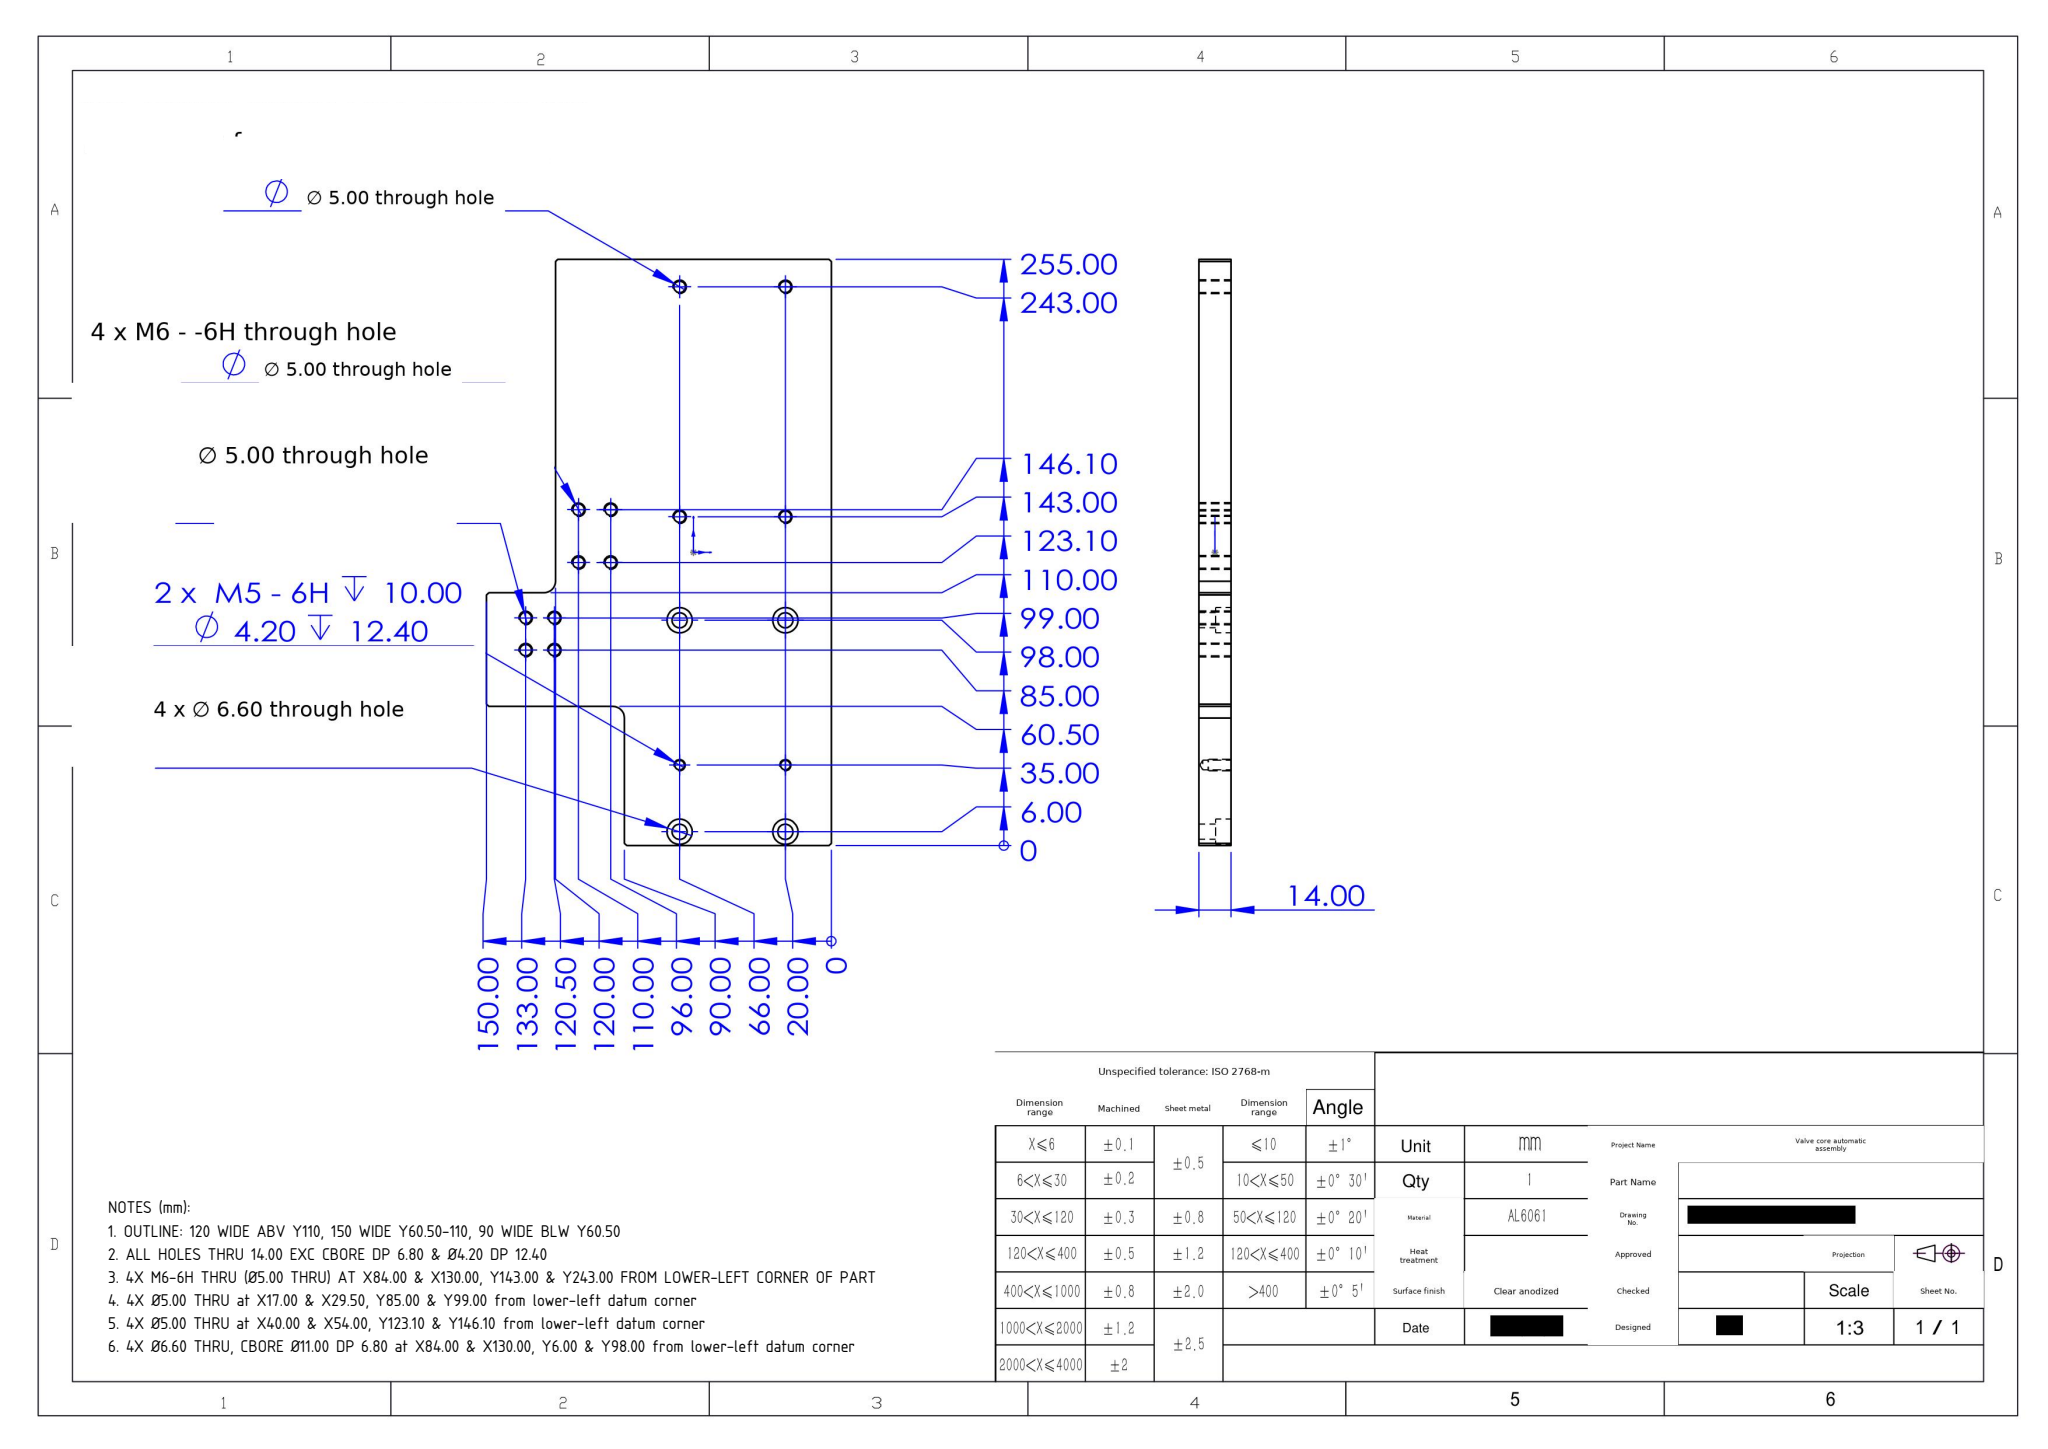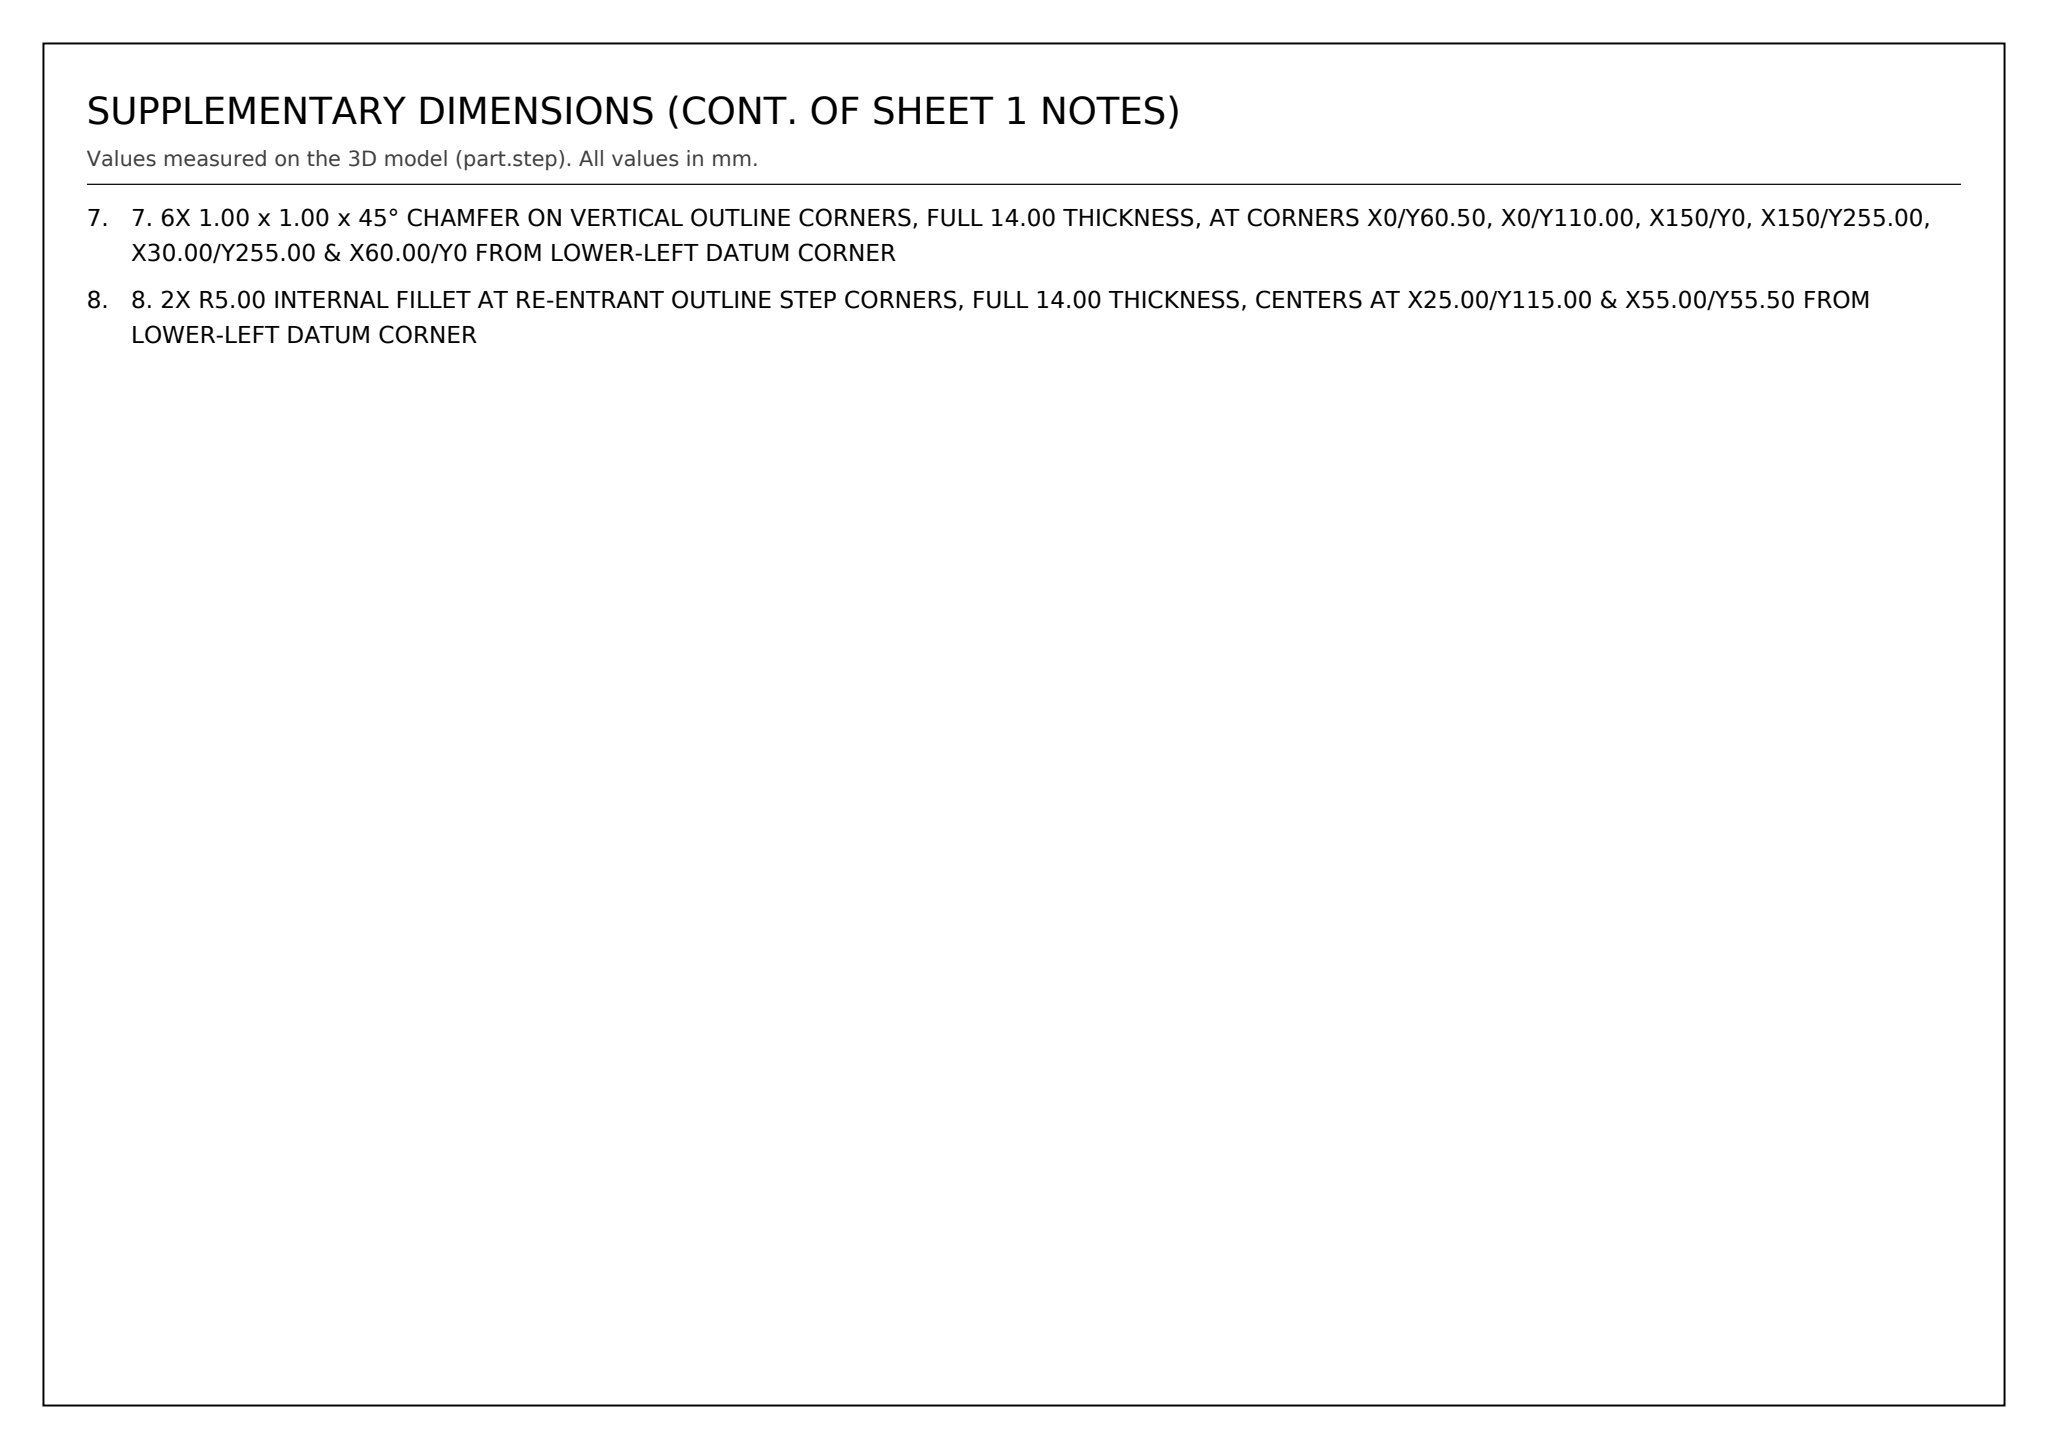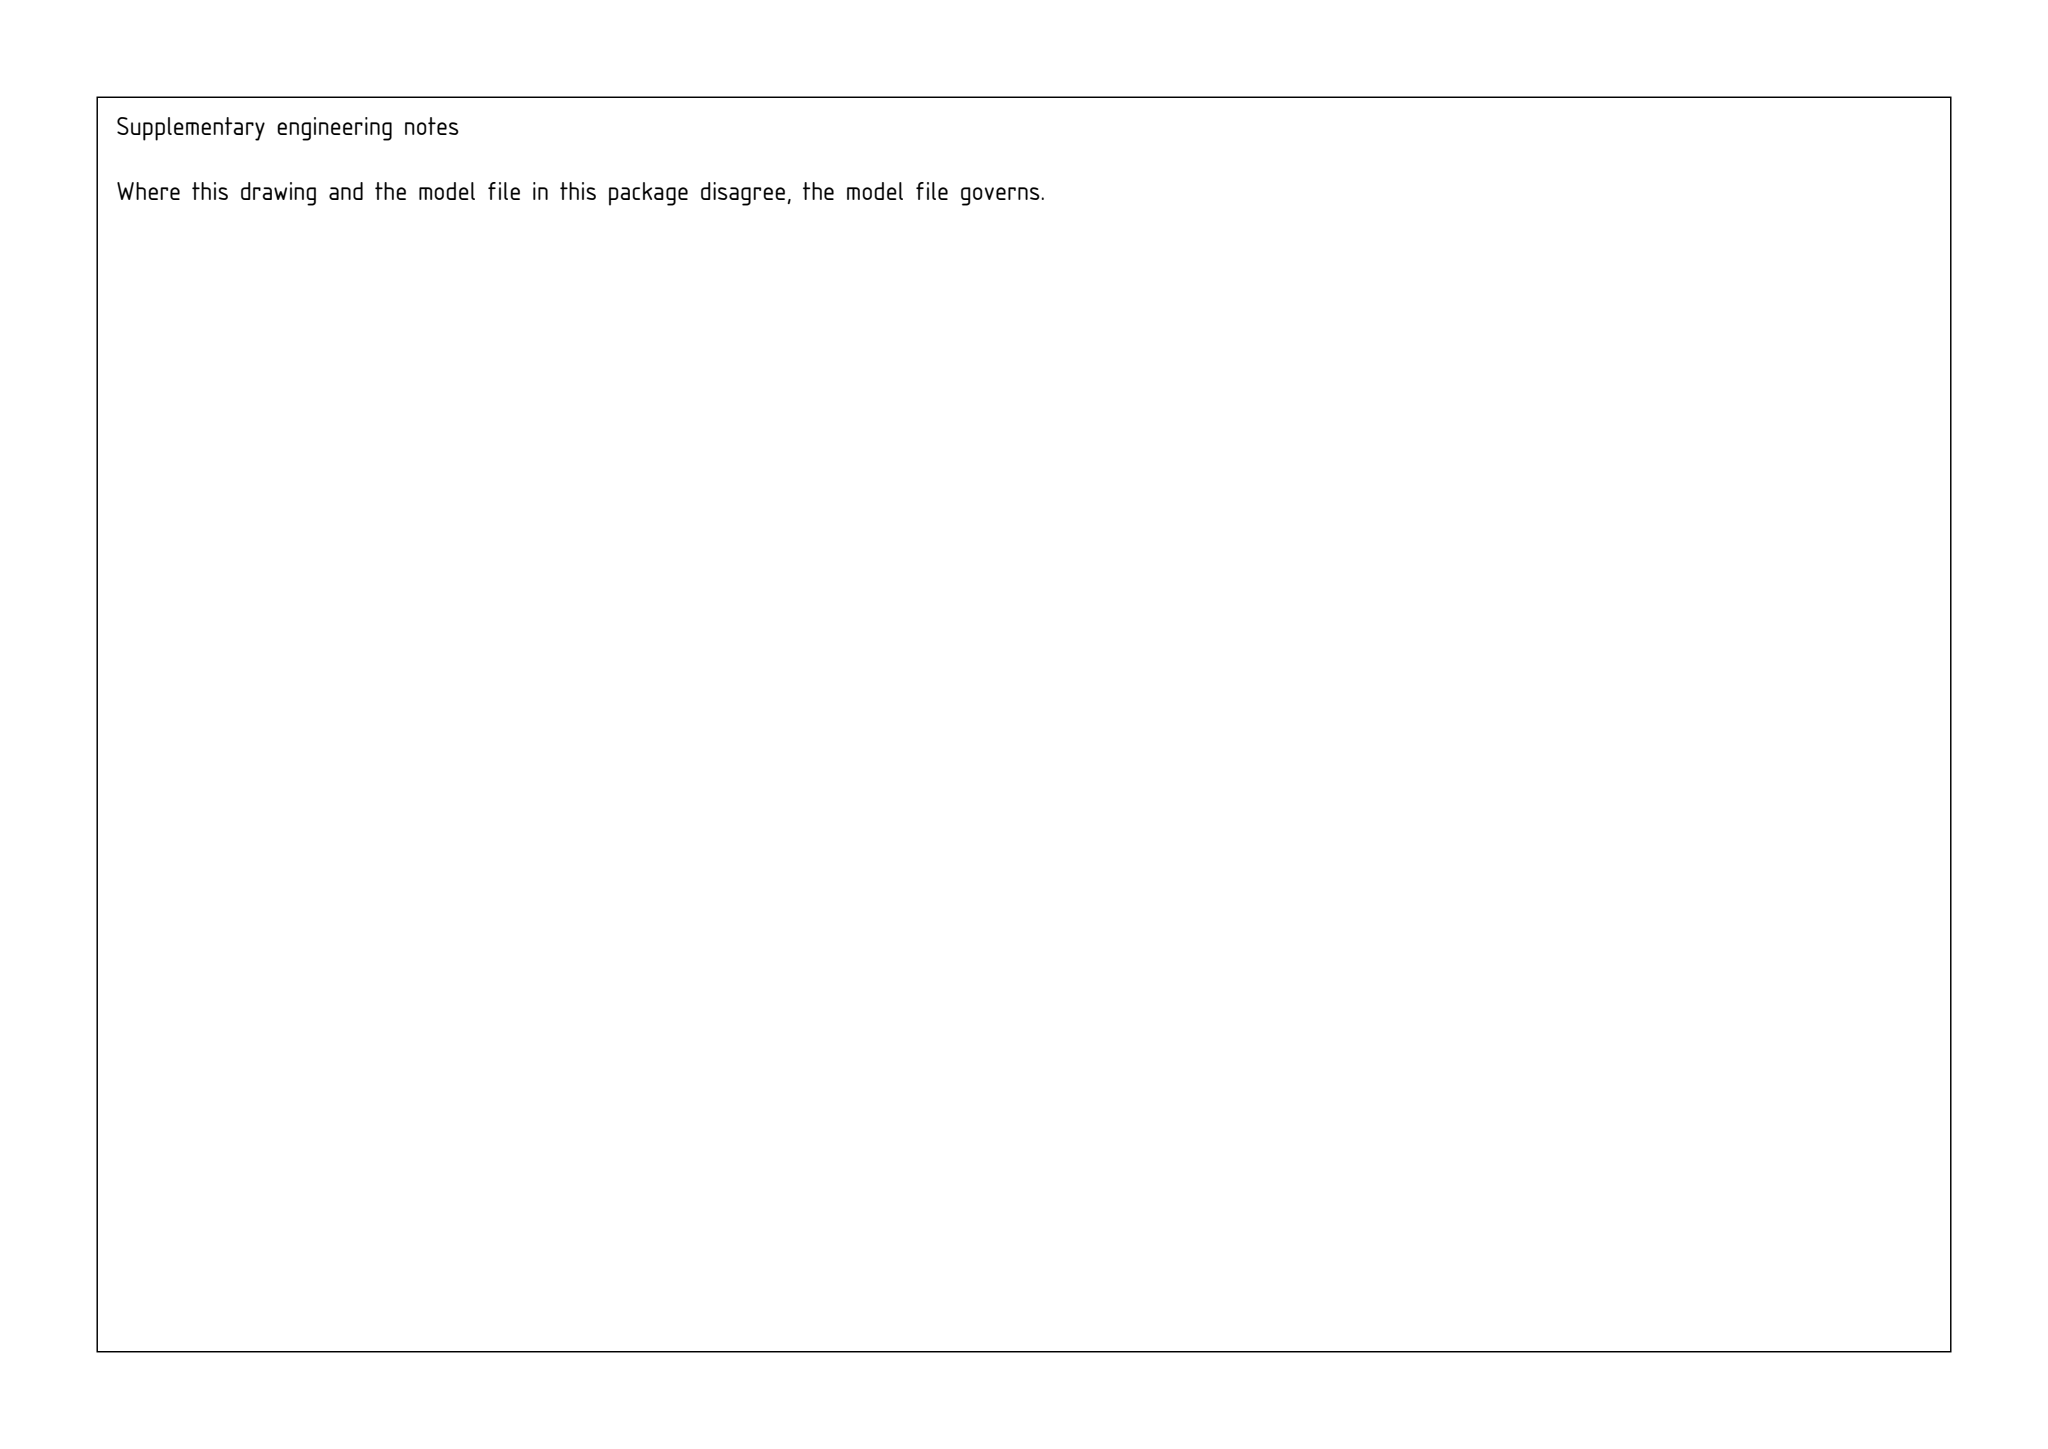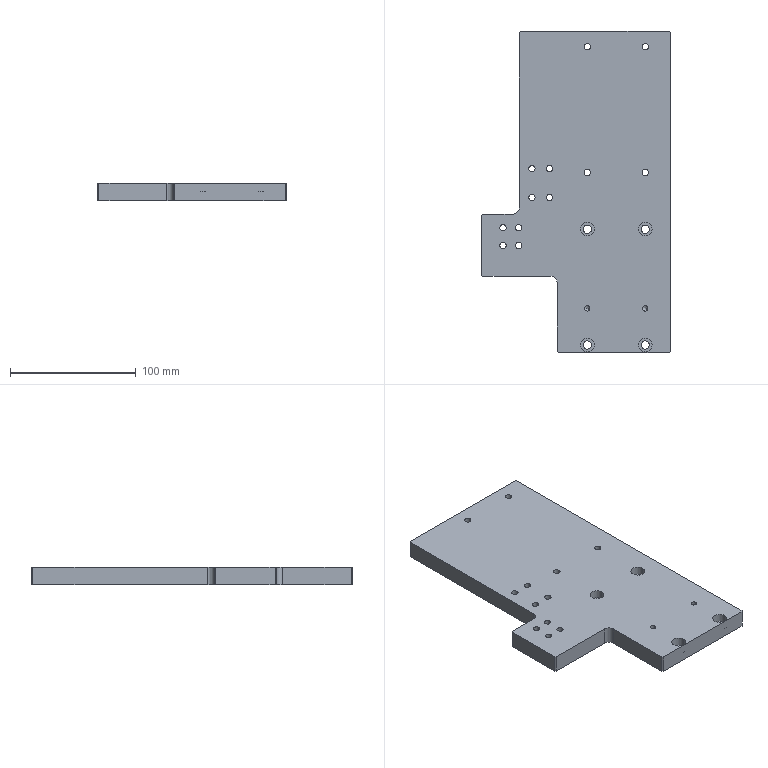Part | SolidWorks | mm | 1 solid | 70 faces | box 150 x 255 x 14 mm | volume 416664 mm3 | cylinder 46 | plane 20 | cone 4 | commonest cylinder face diameters 5 x24 11 x8 6.6 x8 4.2 x4 10 x2
Drawing notes:
OUTLINE: 120 WIDE ABV Y110, 150 WIDE Y60.50-110, 90 WIDE BLW Y60.50 | from the solid: x-planes 0/30/60/150 with y-planes 0/60.5/110/255; steps at x=30 (120 wide) above y110 and x=60 (90 wide) below y60.50
ALL HOLES THRU 14.00 EXC CBORE DP 6.80 & Ø4.20 DP 12.40 | from the solid: Ø5.0 and Ø10.0 cyls L=14.0 full thickness; Ø4.2 cyls L=12.4 blind w/118° pt; Ø11 cbore L=6.8
4X M6-6H THRU (Ø5.00 THRU) AT X84.00 & X130.00, Y143.00 & Y243.00 FROM LOWER-LEFT CORNER OF PART | from the solid: cylinders dia 5.0, axis z, pos (84.0,143.0), (84.0,243.0), (130.0,143.0), (130.0,243.0), length 14.0
4X Ø5.00 THRU at X17.00 & X29.50, Y85.00 & Y99.00 from lower-left datum corner | from the solid: cylinders dia 5.0 axis z at [17,85],[17,99],[29.5,85],[29.5,99], length 14.0
4X Ø5.00 THRU at X40.00 & X54.00, Y123.10 & Y146.10 from lower-left datum corner | from the solid: cylinders dia 5.0 axis z at [40,123.1],[40,146.1],[54,123.1],[54,146.1], length 14.0
4X Ø6.60 THRU, CBORE Ø11.00 DP 6.80 at X84.00 & X130.00, Y6.00 & Y98.00 from lower-left datum corner | from the solid: cylinders dia 6.6 at [84,6],[84,98],[130,6],[130,98] and dia 11.0 same positions length 6.8; plane z=7.2
7. 6X 1.00 x 1.00 x 45° CHAMFER ON VERTICAL OUTLINE CORNERS, FULL 14.00 THICKNESS, AT CORNERS X0/Y60.50, X0/Y110.00, X150/Y0, X150/Y255.00, X30.00/Y255.00 & X60.00/Y0 FROM LOWER-LEFT DATUM CORNER | from the solid: inclined_planes: six 45°/45°/90° faces, size 1.0 x 1.0 x 14.0, bbox_from [0,109,0], [0,60.5,0], [149,0,0], [149,254,0], [30,254,0], [60,0,0]
8. 2X R5.00 INTERNAL FILLET AT RE-ENTRANT OUTLINE STEP CORNERS, FULL 14.00 THICKNESS, CENTERS AT X25.00/Y115.00 & X55.00/Y55.50 FROM LOWER-LEFT DATUM CORNER | from the solid: cylinders: concave arc dia 10.0 (R5.0), axis z at [25.0,115.0] and [55.0,55.5], from z 0.0 to 14.0, arc 90°
build123d program:
from build123d import *

# Parameters (mm, degrees)
SKETCH1_W                                          = 120
SKETCH1_H                                          = 255
BOSS_EXTRUDE1_DEPTH                                = 7
M6_TAPPED_HOLE1_D                                  = 5
HOLE_SIZE_ACCORDING_TO_TYPE_1_OF_HEXAG_D           = 6.6
HOLE_SIZE_ACCORDING_TO_TYPE_1_OF_HEXAG_CBORE_D     = 11
HOLE_SIZE_ACCORDING_TO_TYPE_1_OF_HEXAG_CBORE_DEPTH = 6.8
M6_TAPPED_HOLE2_D                                  = 5
SKETCH10_W                                         = 30
SKETCH10_H                                         = 110
BOSS_EXTRUDE2_DEPTH                                = 14
M6_TAPPED_HOLE3_D                                  = 5
SKETCH13_W                                         = 60
SKETCH13_H                                         = 60.5
CUT_EXTRUDE1_DEPTH                                 = 157.692
FILLET1_R                                          = 5
CHAMFER1_SIZE                                      = 1
M5_TAPPED_HOLE1_D                                  = 4.2
M5_TAPPED_HOLE1_DEPTH                              = 12.4
M5_TAPPED_HOLE1_TIP                                = 1.262


with BuildPart() as part:
    # Sketch1 → Boss-Extrude1 (new, symmetric)
    with BuildSketch(Plane.XY):
        Rectangle(SKETCH1_W, SKETCH1_H)
    extrude(amount=BOSS_EXTRUDE1_DEPTH, both=True)

    # M6 Tapped Hole1 (through all)
    with Locations(Plane(origin=(0, 0, -7), x_dir=(-1, 0, 0), z_dir=(0, 0, -1))):
        with Locations((50, 18.6), (36, -4.4), (50, -4.4), (36, 18.6)):
            Hole(M6_TAPPED_HOLE1_D / 2)

    # Hole Size _According to_ Type 1 of Hexag (through all)
    with Locations(Plane.XY.offset(7)):
        with Locations((-6, -29.5), (40, -121.5), (-6, -121.5), (40, -29.5)):
            CounterBoreHole(HOLE_SIZE_ACCORDING_TO_TYPE_1_OF_HEXAG_D / 2, HOLE_SIZE_ACCORDING_TO_TYPE_1_OF_HEXAG_CBORE_D / 2, HOLE_SIZE_ACCORDING_TO_TYPE_1_OF_HEXAG_CBORE_DEPTH)

    # M6 Tapped Hole2 (through all)
    with Locations(Plane.XY.offset(7)):
        with Locations((-6, 115.5), (40, 15.5), (-6, 15.5), (40, 115.5)):
            Hole(M6_TAPPED_HOLE2_D / 2)

    # Sketch10 → Boss-Extrude2 (add)
    with BuildSketch(Plane.XY.offset(7)):
        with Locations((-75, -72.5)):
            Rectangle(SKETCH10_W, SKETCH10_H)
    extrude(amount=-BOSS_EXTRUDE2_DEPTH)

    # M6 Tapped Hole3 (through all)
    with Locations(Plane.XY.offset(7)):
        with Locations((-73, -28.5), (-60.5, -42.5), (-73, -42.5), (-60.5, -28.5)):
            Hole(M6_TAPPED_HOLE3_D / 2)

    # Sketch13 → Cut-Extrude1 (cut, through all)
    with BuildSketch(Plane.XY.offset(7)):
        with Locations((-60, -97.25)):
            Rectangle(SKETCH13_W, SKETCH13_H)
    extrude(amount=-CUT_EXTRUDE1_DEPTH, mode=Mode.SUBTRACT)

    # Fillet1
    fillet1_edges = [part.edges().sort_by_distance(p)[0] for p in [
        (-60, -17.5, 0),
        (-30, -67, 0),
    ]]
    fillet(fillet1_edges, radius=FILLET1_R)

    # Chamfer1
    chamfer1_edges = [part.edges().sort_by_distance(p)[0] for p in [
        (-90, -17.5, 0),
        (-90, -67, 0),
        (-30, -127.5, 0),
        (60, -127.5, 0),
        (-60, 127.5, 0),
        (60, 127.5, 0),
    ]]
    chamfer(chamfer1_edges, length=CHAMFER1_SIZE)

    # M5 Tapped Hole1
    with Locations(Plane.XY.offset(7)):
        with Locations((40, -92.5), (-6, -92.5)):
            Hole(M5_TAPPED_HOLE1_D / 2, depth=M5_TAPPED_HOLE1_DEPTH)
            with Locations((0, 0, -(M5_TAPPED_HOLE1_DEPTH + M5_TAPPED_HOLE1_TIP / 2))):  # 118° drill point
                Cone(0, M5_TAPPED_HOLE1_D / 2, M5_TAPPED_HOLE1_TIP, mode=Mode.SUBTRACT)


solid = part.part